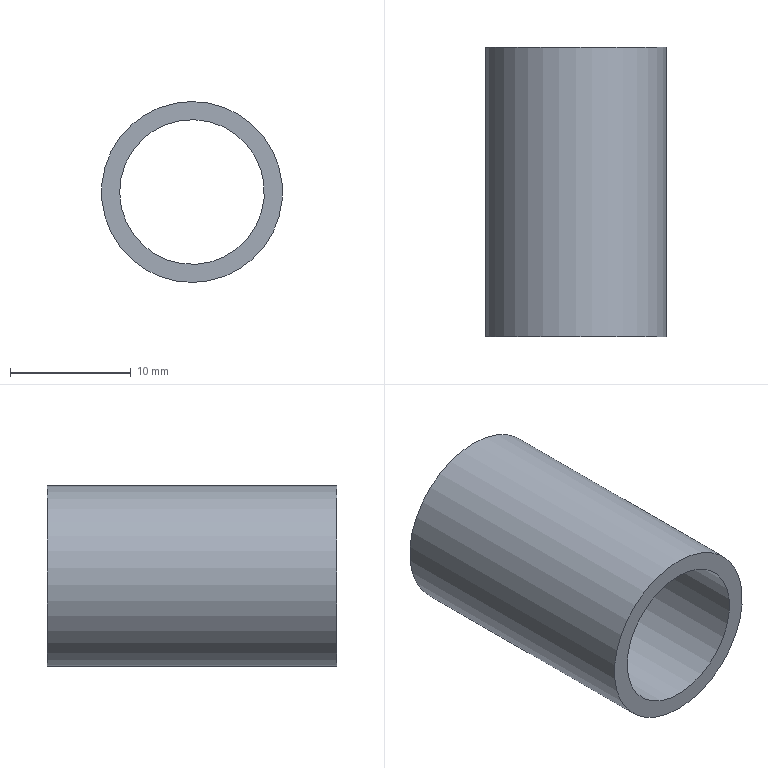Component | NX | ROD_BUSH_LOWER_2 | 1 solid | 4 faces | box 15 x 24 x 15 mm | volume 1527 mm3 | cylinder 2 | plane 2 | commonest cylinder face diameters 15 x1 12 x1
STEP:
#1=CARTESIAN_POINT('',(0.,0.,0.));
#2=DIRECTION('',(0.,0.,1.));
#3=DIRECTION('',(1.,0.,0.));
#4=AXIS2_PLACEMENT_3D('',#1,#2,#3);
#5=CARTESIAN_POINT('',(-29.728,-10.,26.564));
#6=VERTEX_POINT('',#5);
#7=CARTESIAN_POINT('',(-37.198,-10.,27.241));
#8=DIRECTION('',(0.,-1.,0.));
#9=DIRECTION('',(0.9959,0.,-0.09026));
#10=AXIS2_PLACEMENT_3D('',#7,#8,#9);
#11=CIRCLE('',#10,7.5);
#12=CARTESIAN_POINT('',(-37.198,-10.,27.241));
#13=DIRECTION('',(0.,1.,0.));
#14=DIRECTION('',(-0.9959,0.,0.09026));
#15=AXIS2_PLACEMENT_3D('',#12,#13,#14);
#16=CYLINDRICAL_SURFACE('',#15,7.5);
#17=CARTESIAN_POINT('',(9.425,0.));
#18=DIRECTION('',(-1.,0.));
#19=VECTOR('',#18,1.);
#20=LINE('',#17,#19);
#21=(GEOMETRIC_REPRESENTATION_CONTEXT(2)PARAMETRIC_REPRESENTATION_CONTEXT()REPRESENTATION_CONTEXT('',''));
#22=DEFINITIONAL_REPRESENTATION('',(#20),#21);
#23=PCURVE('',#16,#22);
#24=CARTESIAN_POINT('',(-37.198,-10.,27.241));
#25=DIRECTION('',(0.,-1.,0.));
#26=DIRECTION('',(0.9959,0.,-0.09026));
#27=AXIS2_PLACEMENT_3D('',#24,#25,#26);
#28=PLANE('',#27);
#29=CARTESIAN_POINT('',(0.,0.));
#30=DIRECTION('',(1.,-0.));
#31=AXIS2_PLACEMENT_2D('',#29,#30);
#32=CIRCLE('',#31,7.5);
#33=(GEOMETRIC_REPRESENTATION_CONTEXT(2)PARAMETRIC_REPRESENTATION_CONTEXT()REPRESENTATION_CONTEXT('',''));
#34=DEFINITIONAL_REPRESENTATION('',(#32),#33);
#35=PCURVE('',#28,#34);
#36=SURFACE_CURVE('',#11,(#23,#35),.PCURVE_S1.);
#37=EDGE_CURVE('',#6,#6,#36,.T.);
#38=ORIENTED_EDGE('',*,*,#37,.F.);
#39=CARTESIAN_POINT('',(-29.728,14.,26.564));
#40=VERTEX_POINT('',#39);
#41=CARTESIAN_POINT('',(-29.728,-10.,26.564));
#42=CARTESIAN_POINT('',(-29.728,14.,26.564));
#43=B_SPLINE_CURVE_WITH_KNOTS('',1,(#41,#42),.UNSPECIFIED.,.F.,.F.,(2,2),(0.,24.),.PIECEWISE_BEZIER_KNOTS.);
#44=CARTESIAN_POINT('',(9.425,0.));
#45=DIRECTION('',(0.,1.));
#46=VECTOR('',#45,1.);
#47=LINE('',#44,#46);
#48=(GEOMETRIC_REPRESENTATION_CONTEXT(2)PARAMETRIC_REPRESENTATION_CONTEXT()REPRESENTATION_CONTEXT('',''));
#49=DEFINITIONAL_REPRESENTATION('',(#47),#48);
#50=PCURVE('',#16,#49);
#51=CARTESIAN_POINT('',(3.142,0.));
#52=DIRECTION('',(0.,1.));
#53=VECTOR('',#52,1.);
#54=LINE('',#51,#53);
#55=(GEOMETRIC_REPRESENTATION_CONTEXT(2)PARAMETRIC_REPRESENTATION_CONTEXT()REPRESENTATION_CONTEXT('',''));
#56=DEFINITIONAL_REPRESENTATION('',(#54),#55);
#57=PCURVE('',#16,#56);
#58=SEAM_CURVE('',#43,(#50,#57),.PCURVE_S1.);
#59=EDGE_CURVE('',#6,#40,#58,.T.);
#60=ORIENTED_EDGE('',*,*,#59,.T.);
#61=CARTESIAN_POINT('',(-37.198,14.,27.241));
#62=DIRECTION('',(0.,-1.,0.));
#63=DIRECTION('',(0.9959,0.,-0.09026));
#64=AXIS2_PLACEMENT_3D('',#61,#62,#63);
#65=CIRCLE('',#64,7.5);
#66=CARTESIAN_POINT('',(9.425,24.));
#67=DIRECTION('',(-1.,0.));
#68=VECTOR('',#67,1.);
#69=LINE('',#66,#68);
#70=(GEOMETRIC_REPRESENTATION_CONTEXT(2)PARAMETRIC_REPRESENTATION_CONTEXT()REPRESENTATION_CONTEXT('',''));
#71=DEFINITIONAL_REPRESENTATION('',(#69),#70);
#72=PCURVE('',#16,#71);
#73=CARTESIAN_POINT('',(-37.198,14.,27.241));
#74=DIRECTION('',(0.,-1.,0.));
#75=DIRECTION('',(0.9959,0.,-0.09026));
#76=AXIS2_PLACEMENT_3D('',#73,#74,#75);
#77=PLANE('',#76);
#78=CARTESIAN_POINT('',(0.,0.));
#79=DIRECTION('',(1.,-0.));
#80=AXIS2_PLACEMENT_2D('',#78,#79);
#81=CIRCLE('',#80,7.5);
#82=(GEOMETRIC_REPRESENTATION_CONTEXT(2)PARAMETRIC_REPRESENTATION_CONTEXT()REPRESENTATION_CONTEXT('',''));
#83=DEFINITIONAL_REPRESENTATION('',(#81),#82);
#84=PCURVE('',#77,#83);
#85=SURFACE_CURVE('',#65,(#72,#84),.PCURVE_S1.);
#86=EDGE_CURVE('',#40,#40,#85,.T.);
#87=ORIENTED_EDGE('',*,*,#86,.T.);
#88=ORIENTED_EDGE('',*,*,#59,.F.);
#89=EDGE_LOOP('',(#38,#60,#87,#88));
#90=FACE_BOUND('',#89,.T.);
#91=ADVANCED_FACE('',(#90),#16,.T.);
#92=CARTESIAN_POINT('',(-31.222,-10.,26.699));
#93=VERTEX_POINT('',#92);
#94=CARTESIAN_POINT('',(-37.198,-10.,27.241));
#95=DIRECTION('',(0.,-1.,0.));
#96=DIRECTION('',(0.9959,0.,-0.09026));
#97=AXIS2_PLACEMENT_3D('',#94,#95,#96);
#98=CIRCLE('',#97,6.);
#99=CARTESIAN_POINT('',(-37.198,-10.,27.241));
#100=DIRECTION('',(0.,1.,0.));
#101=DIRECTION('',(-0.9959,0.,0.09026));
#102=AXIS2_PLACEMENT_3D('',#99,#100,#101);
#103=CYLINDRICAL_SURFACE('',#102,6.);
#104=CARTESIAN_POINT('',(9.425,0.));
#105=DIRECTION('',(-1.,0.));
#106=VECTOR('',#105,1.);
#107=LINE('',#104,#106);
#108=(GEOMETRIC_REPRESENTATION_CONTEXT(2)PARAMETRIC_REPRESENTATION_CONTEXT()REPRESENTATION_CONTEXT('',''));
#109=DEFINITIONAL_REPRESENTATION('',(#107),#108);
#110=PCURVE('',#103,#109);
#111=CARTESIAN_POINT('',(0.,0.));
#112=DIRECTION('',(1.,0.));
#113=AXIS2_PLACEMENT_2D('',#111,#112);
#114=CIRCLE('',#113,6.);
#115=(GEOMETRIC_REPRESENTATION_CONTEXT(2)PARAMETRIC_REPRESENTATION_CONTEXT()REPRESENTATION_CONTEXT('',''));
#116=DEFINITIONAL_REPRESENTATION('',(#114),#115);
#117=PCURVE('',#28,#116);
#118=SURFACE_CURVE('',#98,(#110,#117),.PCURVE_S1.);
#119=EDGE_CURVE('',#93,#93,#118,.T.);
#120=ORIENTED_EDGE('',*,*,#119,.F.);
#121=CARTESIAN_POINT('',(-31.222,14.,26.699));
#122=VERTEX_POINT('',#121);
#123=CARTESIAN_POINT('',(-31.222,-10.,26.699));
#124=CARTESIAN_POINT('',(-31.222,14.,26.699));
#125=B_SPLINE_CURVE_WITH_KNOTS('',1,(#123,#124),.UNSPECIFIED.,.F.,.F.,(2,2),(0.,24.),.PIECEWISE_BEZIER_KNOTS.);
#126=CARTESIAN_POINT('',(9.425,0.));
#127=DIRECTION('',(0.,1.));
#128=VECTOR('',#127,1.);
#129=LINE('',#126,#128);
#130=(GEOMETRIC_REPRESENTATION_CONTEXT(2)PARAMETRIC_REPRESENTATION_CONTEXT()REPRESENTATION_CONTEXT('',''));
#131=DEFINITIONAL_REPRESENTATION('',(#129),#130);
#132=PCURVE('',#103,#131);
#133=CARTESIAN_POINT('',(3.142,0.));
#134=DIRECTION('',(0.,1.));
#135=VECTOR('',#134,1.);
#136=LINE('',#133,#135);
#137=(GEOMETRIC_REPRESENTATION_CONTEXT(2)PARAMETRIC_REPRESENTATION_CONTEXT()REPRESENTATION_CONTEXT('',''));
#138=DEFINITIONAL_REPRESENTATION('',(#136),#137);
#139=PCURVE('',#103,#138);
#140=SEAM_CURVE('',#125,(#132,#139),.PCURVE_S1.);
#141=EDGE_CURVE('',#93,#122,#140,.T.);
#142=ORIENTED_EDGE('',*,*,#141,.T.);
#143=CARTESIAN_POINT('',(-37.198,14.,27.241));
#144=DIRECTION('',(0.,-1.,0.));
#145=DIRECTION('',(0.9959,0.,-0.09026));
#146=AXIS2_PLACEMENT_3D('',#143,#144,#145);
#147=CIRCLE('',#146,6.);
#148=CARTESIAN_POINT('',(9.425,24.));
#149=DIRECTION('',(-1.,0.));
#150=VECTOR('',#149,1.);
#151=LINE('',#148,#150);
#152=(GEOMETRIC_REPRESENTATION_CONTEXT(2)PARAMETRIC_REPRESENTATION_CONTEXT()REPRESENTATION_CONTEXT('',''));
#153=DEFINITIONAL_REPRESENTATION('',(#151),#152);
#154=PCURVE('',#103,#153);
#155=CARTESIAN_POINT('',(0.,0.));
#156=DIRECTION('',(1.,0.));
#157=AXIS2_PLACEMENT_2D('',#155,#156);
#158=CIRCLE('',#157,6.);
#159=(GEOMETRIC_REPRESENTATION_CONTEXT(2)PARAMETRIC_REPRESENTATION_CONTEXT()REPRESENTATION_CONTEXT('',''));
#160=DEFINITIONAL_REPRESENTATION('',(#158),#159);
#161=PCURVE('',#77,#160);
#162=SURFACE_CURVE('',#147,(#154,#161),.PCURVE_S1.);
#163=EDGE_CURVE('',#122,#122,#162,.T.);
#164=ORIENTED_EDGE('',*,*,#163,.T.);
#165=ORIENTED_EDGE('',*,*,#141,.F.);
#166=EDGE_LOOP('',(#120,#142,#164,#165));
#167=FACE_BOUND('',#166,.F.);
#168=ADVANCED_FACE('',(#167),#103,.F.);
#169=ORIENTED_EDGE('',*,*,#37,.T.);
#170=EDGE_LOOP('',(#169));
#171=FACE_BOUND('',#170,.T.);
#172=ORIENTED_EDGE('',*,*,#119,.F.);
#173=EDGE_LOOP('',(#172));
#174=FACE_BOUND('',#173,.T.);
#175=ADVANCED_FACE('',(#171,#174),#28,.T.);
#176=ORIENTED_EDGE('',*,*,#86,.F.);
#177=EDGE_LOOP('',(#176));
#178=FACE_BOUND('',#177,.T.);
#179=ORIENTED_EDGE('',*,*,#163,.T.);
#180=EDGE_LOOP('',(#179));
#181=FACE_BOUND('',#180,.T.);
#182=ADVANCED_FACE('',(#178,#181),#77,.F.);
#183=CLOSED_SHELL('',(#91,#168,#175,#182));
#184=MANIFOLD_SOLID_BREP('',#183);
#185=(LENGTH_UNIT()NAMED_UNIT(*)SI_UNIT(.MILLI.,.METRE.));
#186=UNCERTAINTY_MEASURE_WITH_UNIT(LENGTH_MEASURE(0.00001),#185,'','');
#187=(NAMED_UNIT(*)PLANE_ANGLE_UNIT()SI_UNIT($,.RADIAN.));
#188=(NAMED_UNIT(*)SI_UNIT($,.STERADIAN.)SOLID_ANGLE_UNIT());
#189=(GEOMETRIC_REPRESENTATION_CONTEXT(3)GLOBAL_UNCERTAINTY_ASSIGNED_CONTEXT((#186))GLOBAL_UNIT_ASSIGNED_CONTEXT((#185,#187,#188))REPRESENTATION_CONTEXT('',''));
#190=ADVANCED_BREP_SHAPE_REPRESENTATION('',(#4,#184),#189);